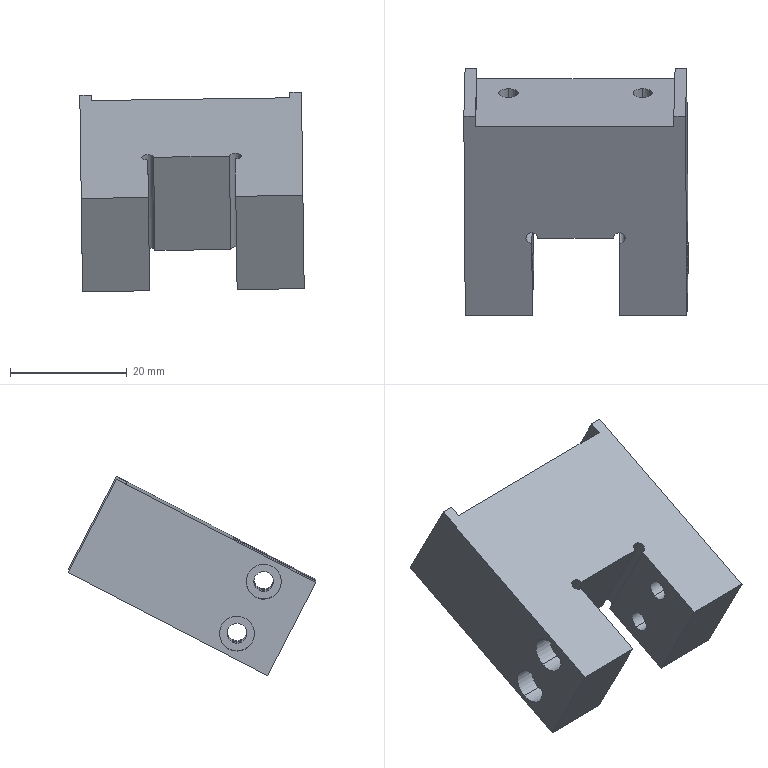Component | SolidWorks | 2018SOLIDWORKS1400000009-1 | 1 solid | 44 faces | box 38.46 x 42.47 x 34.19 mm | volume 20152 mm3 | cylinder 22 | plane 18 | cone 4 | commonest cylinder face diameters 6 x8 3.4 x8 3.3 x4 2 x2 | material 6061 Alloy
build123d program:
from build123d import *

# Parameters (mm, degrees)
SKETCH1_W                                          = 38.5
SKETCH1_H                                          = 38
BOSS_EXTRUDE1_DEPTH                                = 9
SKETCH2_W                                          = 15
SKETCH2_H                                          = 15
CUT_EXTRUDE1_DEPTH                                 = 33.489
SKETCH3_R                                          = 1
CUT_EXTRUDE2_DEPTH                                 = 33.489
HOLE_SIZE_ACCORDING_TO_TYPE_1_OF_HEXAG_D           = 3.4
HOLE_SIZE_ACCORDING_TO_TYPE_1_OF_HEXAG_DEPTH       = 26.499
HOLE_SIZE_ACCORDING_TO_TYPE_1_OF_HEXAG_CBORE_D     = 6
HOLE_SIZE_ACCORDING_TO_TYPE_1_OF_HEXAG_CBORE_DEPTH = 3.4
SKETCH6_W                                          = 18
SKETCH6_H                                          = 34
CUT_EXTRUDE3_DEPTH                                 = 2
M4_TAPPED_HOLE1_D                                  = 3.3
M4_TAPPED_HOLE1_DEPTH                              = 8.1
M4_TAPPED_HOLE1_TIP                                = 0.9914


with BuildPart() as part:
    # Sketch1 → Boss-Extrude1 (new, symmetric)
    with BuildSketch(Plane.XY):
        Rectangle(SKETCH1_W, SKETCH1_H)
    extrude(amount=BOSS_EXTRUDE1_DEPTH, both=True)

    # Sketch2 → Cut-Extrude1 (cut, through all)
    with BuildSketch(Plane.XY.offset(9)):
        with Locations((11.75, 0)):
            Rectangle(SKETCH2_W, SKETCH2_H)
    extrude(amount=-CUT_EXTRUDE1_DEPTH, mode=Mode.SUBTRACT)

    # Sketch3 → Cut-Extrude2 (cut, through all)
    with BuildSketch(Plane.XY.offset(9)):
        with Locations((4.25, -7.5)):
            Circle(SKETCH3_R)
        with Locations((4.25, 7.5)):
            Circle(SKETCH3_R)
    extrude(amount=-CUT_EXTRUDE2_DEPTH, mode=Mode.SUBTRACT)

    # Hole Size _according to_ Type 1 of Hexag
    with Locations(Plane(origin=(0, -19, 0), x_dir=(-1, 0, 0), z_dir=(0, -1, 0))):
        with Locations((-11.25, -5), (-11.25, 5)):
            hole_size_according_to_type_1_of_hexag = CounterBoreHole(HOLE_SIZE_ACCORDING_TO_TYPE_1_OF_HEXAG_D / 2, HOLE_SIZE_ACCORDING_TO_TYPE_1_OF_HEXAG_CBORE_D / 2, HOLE_SIZE_ACCORDING_TO_TYPE_1_OF_HEXAG_CBORE_DEPTH, depth=HOLE_SIZE_ACCORDING_TO_TYPE_1_OF_HEXAG_DEPTH)

    # Mirror1: Hole Size _according to_ Type 1 of Hexag across plane
    add(hole_size_according_to_type_1_of_hexag.mirror(Plane.ZX), mode=Mode.SUBTRACT)

    # Sketch6 → Cut-Extrude3 (cut)
    with BuildSketch(Plane.ZY.offset(19.25)):
        Rectangle(SKETCH6_W, SKETCH6_H)
    extrude(amount=-CUT_EXTRUDE3_DEPTH, mode=Mode.SUBTRACT)

    # M4 Tapped Hole1
    with Locations(Plane.ZY.offset(17.25)):
        with Locations((-3.5, 11.5), (-3.5, -11.5)):
            Hole(M4_TAPPED_HOLE1_D / 2, depth=M4_TAPPED_HOLE1_DEPTH)
            with Locations((0, 0, -(M4_TAPPED_HOLE1_DEPTH + M4_TAPPED_HOLE1_TIP / 2))):  # 118° drill point
                Cone(0, M4_TAPPED_HOLE1_D / 2, M4_TAPPED_HOLE1_TIP, mode=Mode.SUBTRACT)


solid = part.part

# Placed as in the assembly
solid = solid.moved(Location((97.53, -54.79, 117.783), (27.325, -0.7042, -89.636)))